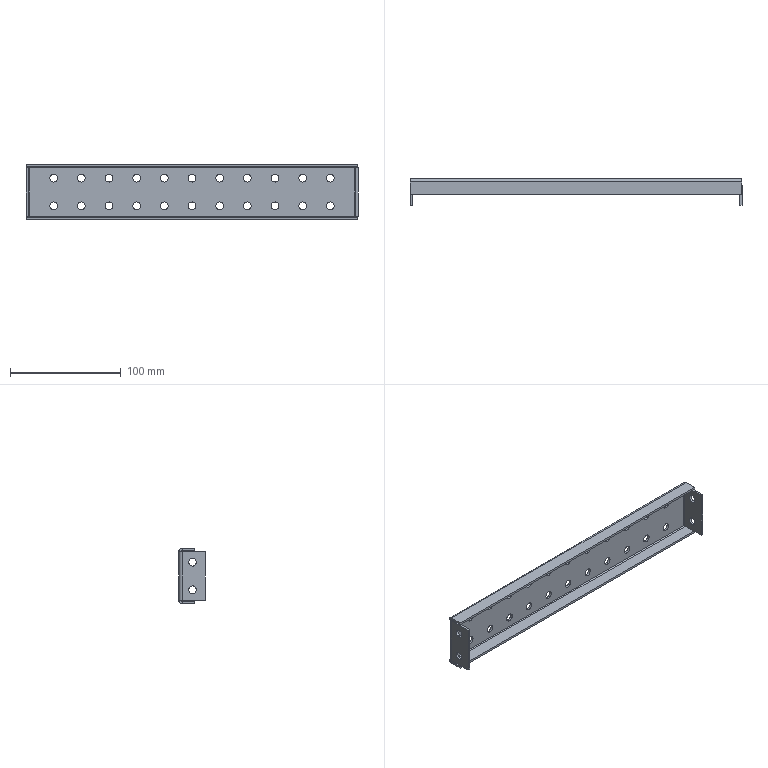Component | SolidWorks | Beam(No.20)-1 | 1 solid | 94 faces | volume 45090 mm3 | cylinder 60 | plane 34 | commonest cylinder face diameters 7 x52 6 x4 2 x4